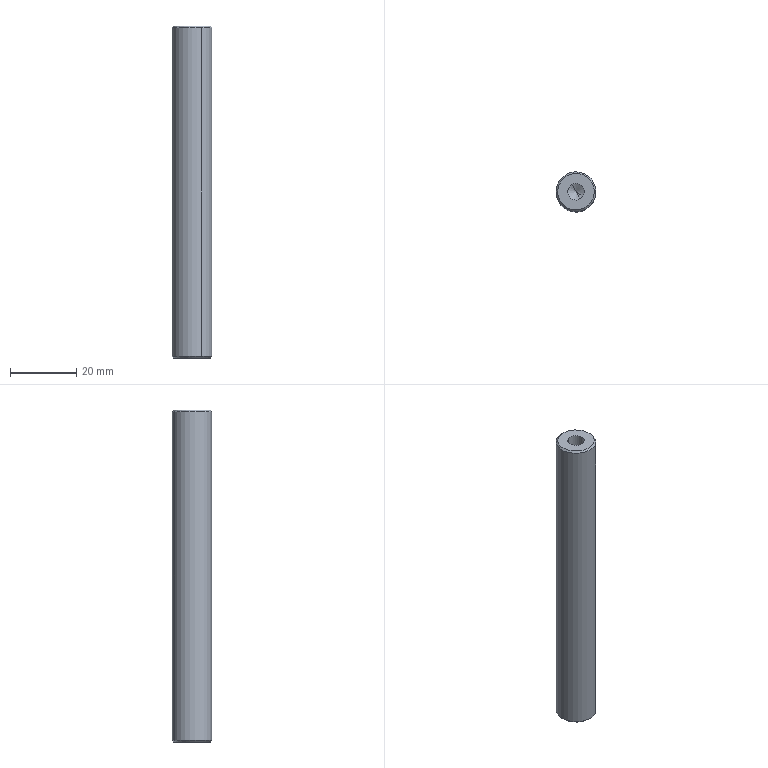Component | SolidWorks | A-C14LocatingMechanismGuidePost-1 | 1 solid | 12 faces | box 12 x 12 x 100 mm | volume 10996 mm3 | cone 6 | cylinder 4 | plane 2 | commonest cylinder face diameters 5 x2 12 x2
build123d program:
from build123d import *

# Parameters (mm, degrees)
SKETCH1_R             = 6
EXTRUDE1_DEPTH        = 100
CHAMFER1_SIZE         = 0.5
M6_TAPPED_HOLE1_D     = 5
M6_TAPPED_HOLE1_DEPTH = 15
M6_TAPPED_HOLE1_TIP   = 1.502


with BuildPart() as part:
    # Sketch1 → Extrude1 (new body)
    with BuildSketch(Plane.XY):
        Circle(SKETCH1_R)
    extrude(amount=EXTRUDE1_DEPTH)

    # Chamfer1
    chamfer1_edges = [part.edges().sort_by_distance(p)[0] for p in [
        (-6, 0, 0),
        (-6, 0, 100),
    ]]
    chamfer(chamfer1_edges, length=CHAMFER1_SIZE)

    # M6 Tapped Hole1
    with Locations(Plane(origin=(0, 0, 0), x_dir=(-1, 0, 0), z_dir=(0, 0, -1))):
        with Locations((0, 0)):
            Hole(M6_TAPPED_HOLE1_D / 2, depth=M6_TAPPED_HOLE1_DEPTH)
            with Locations((0, 0, -(M6_TAPPED_HOLE1_DEPTH + M6_TAPPED_HOLE1_TIP / 2))):  # 118° drill point
                Cone(0, M6_TAPPED_HOLE1_D / 2, M6_TAPPED_HOLE1_TIP, mode=Mode.SUBTRACT)


solid = part.part

# Placed as in the assembly
solid = solid.moved(Location((-53.181, -42.432, 18), (180, 0, 0)))
STEP:
#1=COLOUR_RGB('',0.7922,0.8196,0.9333);
#2=FILL_AREA_STYLE_COLOUR('',#1);
#3=FILL_AREA_STYLE('',(#2));
#4=SURFACE_STYLE_FILL_AREA(#3);
#5=SURFACE_SIDE_STYLE('',(#4));
#6=SURFACE_STYLE_USAGE(.BOTH.,#5);
#7=PRESENTATION_STYLE_ASSIGNMENT((#6));
#8=CARTESIAN_POINT('',(-2.142,-1.585,0.1181));
#9=VERTEX_POINT('',#8);
#10=CARTESIAN_POINT('',(-2.046,-1.757,0.1181));
#11=VERTEX_POINT('',#10);
#12=CARTESIAN_POINT('',(-2.094,-1.671,0.1181));
#13=DIRECTION('',(-0.,0.,1.));
#14=DIRECTION('',(0.4859,-0.874,0.));
#15=AXIS2_PLACEMENT_3D('',#12,#13,#14);
#16=CIRCLE('',#15,0.09843);
#17=EDGE_CURVE('',#9,#11,#16,.T.);
#18=ORIENTED_EDGE('',*,*,#17,.F.);
#19=CARTESIAN_POINT('',(-2.142,-1.585,0.7087));
#20=VERTEX_POINT('',#19);
#21=CARTESIAN_POINT('',(-2.142,-1.585,0.7087));
#22=DIRECTION('',(-0.,0.,1.));
#23=VECTOR('',#22,39.37);
#24=LINE('',#21,#23);
#25=EDGE_CURVE('',#9,#20,#24,.T.);
#26=ORIENTED_EDGE('',*,*,#25,.T.);
#27=CARTESIAN_POINT('',(-2.046,-1.757,0.7087));
#28=VERTEX_POINT('',#27);
#29=CARTESIAN_POINT('',(-2.094,-1.671,0.7087));
#30=DIRECTION('',(-0.,0.,1.));
#31=DIRECTION('',(0.4859,-0.874,0.));
#32=AXIS2_PLACEMENT_3D('',#29,#30,#31);
#33=CIRCLE('',#32,0.09843);
#34=EDGE_CURVE('',#20,#28,#33,.T.);
#35=ORIENTED_EDGE('',*,*,#34,.T.);
#36=CARTESIAN_POINT('',(-2.046,-1.757,0.7087));
#37=DIRECTION('',(-0.,0.,1.));
#38=VECTOR('',#37,39.37);
#39=LINE('',#36,#38);
#40=EDGE_CURVE('',#11,#28,#39,.T.);
#41=ORIENTED_EDGE('',*,*,#40,.F.);
#42=EDGE_LOOP('',(#18,#26,#35,#41));
#43=FACE_OUTER_BOUND('',#42,.T.);
#44=CARTESIAN_POINT('',(-2.094,-1.671,0.7087));
#45=DIRECTION('',(-0.,0.,1.));
#46=DIRECTION('',(0.4859,-0.874,0.));
#47=AXIS2_PLACEMENT_3D('',#44,#45,#46);
#48=CYLINDRICAL_SURFACE('',#47,0.09843);
#49=ADVANCED_FACE('',(#43),#48,.F.);
#50=CARTESIAN_POINT('',(-2.094,-1.671,0.05897));
#51=VERTEX_POINT('',#50);
#52=CARTESIAN_POINT('',(-2.046,-1.757,0.1181));
#53=DIRECTION('',(0.4165,-0.7492,0.515));
#54=VECTOR('',#53,39.37);
#55=LINE('',#52,#54);
#56=EDGE_CURVE('',#51,#11,#55,.T.);
#57=ORIENTED_EDGE('',*,*,#56,.F.);
#58=CARTESIAN_POINT('',(-2.142,-1.585,0.1181));
#59=DIRECTION('',(-0.4165,0.7492,0.515));
#60=VECTOR('',#59,39.37);
#61=LINE('',#58,#60);
#62=EDGE_CURVE('',#51,#9,#61,.T.);
#63=ORIENTED_EDGE('',*,*,#62,.T.);
#64=ORIENTED_EDGE('',*,*,#17,.T.);
#65=EDGE_LOOP('',(#57,#63,#64));
#66=FACE_OUTER_BOUND('',#65,.T.);
#67=CARTESIAN_POINT('',(-2.094,-1.671,0.1181));
#68=DIRECTION('',(-0.,0.,1.));
#69=DIRECTION('',(0.4859,-0.874,0.));
#70=AXIS2_PLACEMENT_3D('',#67,#68,#69);
#71=CONICAL_SURFACE('',#70,0.09843,1.03);
#72=ADVANCED_FACE('',(#66),#71,.F.);
#73=CARTESIAN_POINT('',(-2.199,-1.481,-3.228));
#74=VERTEX_POINT('',#73);
#75=CARTESIAN_POINT('',(-1.989,-1.86,-3.228));
#76=VERTEX_POINT('',#75);
#77=CARTESIAN_POINT('',(-2.094,-1.671,-3.228));
#78=DIRECTION('',(0.,-0.,-1.));
#79=DIRECTION('',(-0.4859,0.874,0.));
#80=AXIS2_PLACEMENT_3D('',#77,#78,#79);
#81=CIRCLE('',#80,0.2165);
#82=EDGE_CURVE('',#74,#76,#81,.T.);
#83=ORIENTED_EDGE('',*,*,#82,.F.);
#84=CARTESIAN_POINT('',(-2.208,-1.464,-3.209));
#85=VERTEX_POINT('',#84);
#86=CARTESIAN_POINT('',(-2.199,-1.481,-3.228));
#87=DIRECTION('',(-0.3436,0.618,0.7071));
#88=VECTOR('',#87,39.37);
#89=LINE('',#86,#88);
#90=EDGE_CURVE('',#74,#85,#89,.T.);
#91=ORIENTED_EDGE('',*,*,#90,.T.);
#92=CARTESIAN_POINT('',(-1.979,-1.877,-3.209));
#93=VERTEX_POINT('',#92);
#94=CARTESIAN_POINT('',(-2.094,-1.671,-3.209));
#95=DIRECTION('',(-0.,0.,1.));
#96=DIRECTION('',(-0.4859,0.874,0.));
#97=AXIS2_PLACEMENT_3D('',#94,#95,#96);
#98=CIRCLE('',#97,0.2362);
#99=EDGE_CURVE('',#93,#85,#98,.T.);
#100=ORIENTED_EDGE('',*,*,#99,.F.);
#101=CARTESIAN_POINT('',(-1.989,-1.86,-3.228));
#102=DIRECTION('',(0.3436,-0.618,0.7071));
#103=VECTOR('',#102,39.37);
#104=LINE('',#101,#103);
#105=EDGE_CURVE('',#76,#93,#104,.T.);
#106=ORIENTED_EDGE('',*,*,#105,.F.);
#107=EDGE_LOOP('',(#83,#91,#100,#106));
#108=FACE_OUTER_BOUND('',#107,.T.);
#109=CARTESIAN_POINT('',(-2.094,-1.671,-3.228));
#110=DIRECTION('',(-0.,0.,1.));
#111=DIRECTION('',(0.4859,-0.874,0.));
#112=AXIS2_PLACEMENT_3D('',#109,#110,#111);
#113=CONICAL_SURFACE('',#112,0.2165,0.7854);
#114=ADVANCED_FACE('',(#108),#113,.T.);
#115=CARTESIAN_POINT('',(-1.989,-1.86,0.7087));
#116=VERTEX_POINT('',#115);
#117=CARTESIAN_POINT('',(-2.199,-1.481,0.7087));
#118=VERTEX_POINT('',#117);
#119=CARTESIAN_POINT('',(-2.094,-1.671,0.7087));
#120=DIRECTION('',(-0.,0.,1.));
#121=DIRECTION('',(-0.4859,0.874,0.));
#122=AXIS2_PLACEMENT_3D('',#119,#120,#121);
#123=CIRCLE('',#122,0.2165);
#124=EDGE_CURVE('',#116,#118,#123,.T.);
#125=ORIENTED_EDGE('',*,*,#124,.F.);
#126=CARTESIAN_POINT('',(-1.979,-1.877,0.689));
#127=VERTEX_POINT('',#126);
#128=CARTESIAN_POINT('',(-1.979,-1.877,0.689));
#129=DIRECTION('',(0.3436,-0.618,-0.7071));
#130=VECTOR('',#129,39.37);
#131=LINE('',#128,#130);
#132=EDGE_CURVE('',#116,#127,#131,.T.);
#133=ORIENTED_EDGE('',*,*,#132,.T.);
#134=CARTESIAN_POINT('',(-2.208,-1.464,0.689));
#135=VERTEX_POINT('',#134);
#136=CARTESIAN_POINT('',(-2.094,-1.671,0.689));
#137=DIRECTION('',(0.,-0.,-1.));
#138=DIRECTION('',(-0.4859,0.874,0.));
#139=AXIS2_PLACEMENT_3D('',#136,#137,#138);
#140=CIRCLE('',#139,0.2362);
#141=EDGE_CURVE('',#135,#127,#140,.T.);
#142=ORIENTED_EDGE('',*,*,#141,.F.);
#143=CARTESIAN_POINT('',(-2.208,-1.464,0.689));
#144=DIRECTION('',(-0.3436,0.618,-0.7071));
#145=VECTOR('',#144,39.37);
#146=LINE('',#143,#145);
#147=EDGE_CURVE('',#118,#135,#146,.T.);
#148=ORIENTED_EDGE('',*,*,#147,.F.);
#149=EDGE_LOOP('',(#125,#133,#142,#148));
#150=FACE_OUTER_BOUND('',#149,.T.);
#151=CARTESIAN_POINT('',(-2.094,-1.671,0.689));
#152=DIRECTION('',(0.,-0.,-1.));
#153=DIRECTION('',(-0.4859,0.874,0.));
#154=AXIS2_PLACEMENT_3D('',#151,#152,#153);
#155=CONICAL_SURFACE('',#154,0.2362,0.7854);
#156=ADVANCED_FACE('',(#150),#155,.T.);
#157=ORIENTED_EDGE('',*,*,#99,.T.);
#158=CARTESIAN_POINT('',(-2.208,-1.464,-3.228));
#159=DIRECTION('',(-0.,0.,1.));
#160=VECTOR('',#159,39.37);
#161=LINE('',#158,#160);
#162=EDGE_CURVE('',#85,#135,#161,.T.);
#163=ORIENTED_EDGE('',*,*,#162,.T.);
#164=ORIENTED_EDGE('',*,*,#141,.T.);
#165=CARTESIAN_POINT('',(-1.979,-1.877,-3.228));
#166=DIRECTION('',(-0.,0.,1.));
#167=VECTOR('',#166,39.37);
#168=LINE('',#165,#167);
#169=EDGE_CURVE('',#93,#127,#168,.T.);
#170=ORIENTED_EDGE('',*,*,#169,.F.);
#171=EDGE_LOOP('',(#157,#163,#164,#170));
#172=FACE_OUTER_BOUND('',#171,.T.);
#173=CARTESIAN_POINT('',(-2.094,-1.671,-3.228));
#174=DIRECTION('',(-0.,0.,1.));
#175=DIRECTION('',(0.4859,-0.874,0.));
#176=AXIS2_PLACEMENT_3D('',#173,#174,#175);
#177=CYLINDRICAL_SURFACE('',#176,0.2362);
#178=ADVANCED_FACE('',(#172),#177,.T.);
#179=ORIENTED_EDGE('',*,*,#162,.F.);
#180=CARTESIAN_POINT('',(-2.094,-1.671,-3.209));
#181=DIRECTION('',(-0.,0.,1.));
#182=DIRECTION('',(-0.4859,0.874,0.));
#183=AXIS2_PLACEMENT_3D('',#180,#181,#182);
#184=CIRCLE('',#183,0.2362);
#185=EDGE_CURVE('',#85,#93,#184,.T.);
#186=ORIENTED_EDGE('',*,*,#185,.T.);
#187=ORIENTED_EDGE('',*,*,#169,.T.);
#188=CARTESIAN_POINT('',(-2.094,-1.671,0.689));
#189=DIRECTION('',(0.,-0.,-1.));
#190=DIRECTION('',(-0.4859,0.874,0.));
#191=AXIS2_PLACEMENT_3D('',#188,#189,#190);
#192=CIRCLE('',#191,0.2362);
#193=EDGE_CURVE('',#127,#135,#192,.T.);
#194=ORIENTED_EDGE('',*,*,#193,.T.);
#195=EDGE_LOOP('',(#179,#186,#187,#194));
#196=FACE_OUTER_BOUND('',#195,.T.);
#197=CARTESIAN_POINT('',(-2.094,-1.671,-3.228));
#198=DIRECTION('',(-0.,0.,1.));
#199=DIRECTION('',(0.4859,-0.874,0.));
#200=AXIS2_PLACEMENT_3D('',#197,#198,#199);
#201=CYLINDRICAL_SURFACE('',#200,0.2362);
#202=ADVANCED_FACE('',(#196),#201,.T.);
#203=CARTESIAN_POINT('',(-2.094,-1.671,-3.228));
#204=DIRECTION('',(0.,-0.,-1.));
#205=DIRECTION('',(-0.4859,0.874,0.));
#206=AXIS2_PLACEMENT_3D('',#203,#204,#205);
#207=CIRCLE('',#206,0.2165);
#208=EDGE_CURVE('',#76,#74,#207,.T.);
#209=ORIENTED_EDGE('',*,*,#208,.T.);
#210=ORIENTED_EDGE('',*,*,#82,.T.);
#211=EDGE_LOOP('',(#209,#210));
#212=FACE_OUTER_BOUND('',#211,.T.);
#213=CARTESIAN_POINT('',(-2.094,-1.671,-3.228));
#214=DIRECTION('',(0.,-0.,-1.));
#215=DIRECTION('',(-0.4859,0.874,-0.));
#216=AXIS2_PLACEMENT_3D('',#213,#214,#215);
#217=PLANE('',#216);
#218=ADVANCED_FACE('',(#212),#217,.T.);
#219=CARTESIAN_POINT('',(-2.094,-1.671,0.7087));
#220=DIRECTION('',(-0.,0.,1.));
#221=DIRECTION('',(0.4859,-0.874,0.));
#222=AXIS2_PLACEMENT_3D('',#219,#220,#221);
#223=CIRCLE('',#222,0.09843);
#224=EDGE_CURVE('',#28,#20,#223,.T.);
#225=ORIENTED_EDGE('',*,*,#224,.F.);
#226=ORIENTED_EDGE('',*,*,#34,.F.);
#227=EDGE_LOOP('',(#225,#226));
#228=FACE_BOUND('',#227,.T.);
#229=CARTESIAN_POINT('',(-2.094,-1.671,0.7087));
#230=DIRECTION('',(-0.,0.,1.));
#231=DIRECTION('',(-0.4859,0.874,0.));
#232=AXIS2_PLACEMENT_3D('',#229,#230,#231);
#233=CIRCLE('',#232,0.2165);
#234=EDGE_CURVE('',#118,#116,#233,.T.);
#235=ORIENTED_EDGE('',*,*,#234,.T.);
#236=ORIENTED_EDGE('',*,*,#124,.T.);
#237=EDGE_LOOP('',(#235,#236));
#238=FACE_OUTER_BOUND('',#237,.T.);
#239=CARTESIAN_POINT('',(-2.094,-1.671,0.7087));
#240=DIRECTION('',(0.,-0.,-1.));
#241=DIRECTION('',(-0.4859,0.874,-0.));
#242=AXIS2_PLACEMENT_3D('',#239,#240,#241);
#243=PLANE('',#242);
#244=ADVANCED_FACE('',(#228,#238),#243,.F.);
#245=ORIENTED_EDGE('',*,*,#132,.F.);
#246=ORIENTED_EDGE('',*,*,#234,.F.);
#247=ORIENTED_EDGE('',*,*,#147,.T.);
#248=ORIENTED_EDGE('',*,*,#193,.F.);
#249=EDGE_LOOP('',(#245,#246,#247,#248));
#250=FACE_OUTER_BOUND('',#249,.T.);
#251=CARTESIAN_POINT('',(-2.094,-1.671,0.689));
#252=DIRECTION('',(0.,-0.,-1.));
#253=DIRECTION('',(-0.4859,0.874,0.));
#254=AXIS2_PLACEMENT_3D('',#251,#252,#253);
#255=CONICAL_SURFACE('',#254,0.2362,0.7854);
#256=ADVANCED_FACE('',(#250),#255,.T.);
#257=ORIENTED_EDGE('',*,*,#90,.F.);
#258=ORIENTED_EDGE('',*,*,#208,.F.);
#259=ORIENTED_EDGE('',*,*,#105,.T.);
#260=ORIENTED_EDGE('',*,*,#185,.F.);
#261=EDGE_LOOP('',(#257,#258,#259,#260));
#262=FACE_OUTER_BOUND('',#261,.T.);
#263=CARTESIAN_POINT('',(-2.094,-1.671,-3.228));
#264=DIRECTION('',(-0.,0.,1.));
#265=DIRECTION('',(0.4859,-0.874,0.));
#266=AXIS2_PLACEMENT_3D('',#263,#264,#265);
#267=CONICAL_SURFACE('',#266,0.2165,0.7854);
#268=ADVANCED_FACE('',(#262),#267,.T.);
#269=ORIENTED_EDGE('',*,*,#62,.F.);
#270=ORIENTED_EDGE('',*,*,#56,.T.);
#271=CARTESIAN_POINT('',(-2.094,-1.671,0.1181));
#272=DIRECTION('',(-0.,0.,1.));
#273=DIRECTION('',(0.4859,-0.874,0.));
#274=AXIS2_PLACEMENT_3D('',#271,#272,#273);
#275=CIRCLE('',#274,0.09843);
#276=EDGE_CURVE('',#11,#9,#275,.T.);
#277=ORIENTED_EDGE('',*,*,#276,.T.);
#278=EDGE_LOOP('',(#269,#270,#277));
#279=FACE_OUTER_BOUND('',#278,.T.);
#280=CARTESIAN_POINT('',(-2.094,-1.671,0.1181));
#281=DIRECTION('',(-0.,0.,1.));
#282=DIRECTION('',(0.4859,-0.874,0.));
#283=AXIS2_PLACEMENT_3D('',#280,#281,#282);
#284=CONICAL_SURFACE('',#283,0.09843,1.03);
#285=ADVANCED_FACE('',(#279),#284,.F.);
#286=ORIENTED_EDGE('',*,*,#25,.F.);
#287=ORIENTED_EDGE('',*,*,#276,.F.);
#288=ORIENTED_EDGE('',*,*,#40,.T.);
#289=ORIENTED_EDGE('',*,*,#224,.T.);
#290=EDGE_LOOP('',(#286,#287,#288,#289));
#291=FACE_OUTER_BOUND('',#290,.T.);
#292=CARTESIAN_POINT('',(-2.094,-1.671,0.7087));
#293=DIRECTION('',(-0.,0.,1.));
#294=DIRECTION('',(0.4859,-0.874,0.));
#295=AXIS2_PLACEMENT_3D('',#292,#293,#294);
#296=CYLINDRICAL_SURFACE('',#295,0.09843);
#297=ADVANCED_FACE('',(#291),#296,.F.);
#298=CLOSED_SHELL('',(#49,#72,#114,#156,#178,#202,#218,#244,#256,#268,#285,#297));
#299=MANIFOLD_SOLID_BREP('',#298);
#300=STYLED_ITEM('',(#7),#299);
#301=PRESENTATION_LAYER_ASSIGNMENT('','',(#300));
#302=(LENGTH_UNIT()NAMED_UNIT(*)SI_UNIT($,.METRE.));
#303=LENGTH_MEASURE_WITH_UNIT(LENGTH_MEASURE(0.0254),#302);
#304=DIMENSIONAL_EXPONENTS(1.,0.,0.,0.,0.,0.,0.);
#305=(CONVERSION_BASED_UNIT('',#303)LENGTH_UNIT()NAMED_UNIT(#304));
#306=UNCERTAINTY_MEASURE_WITH_UNIT(LENGTH_MEASURE(0.00001),#305,'','');
#307=(NAMED_UNIT(*)PLANE_ANGLE_UNIT()SI_UNIT($,.RADIAN.));
#308=(NAMED_UNIT(*)SI_UNIT($,.STERADIAN.)SOLID_ANGLE_UNIT());
#309=(GEOMETRIC_REPRESENTATION_CONTEXT(3)GLOBAL_UNCERTAINTY_ASSIGNED_CONTEXT((#306))GLOBAL_UNIT_ASSIGNED_CONTEXT((#305,#307,#308))REPRESENTATION_CONTEXT('',''));
#310=MECHANICAL_DESIGN_GEOMETRIC_PRESENTATION_REPRESENTATION('',(#300),#309);
#311=CARTESIAN_POINT('',(0.,0.,0.));
#312=DIRECTION('',(0.,0.,1.));
#313=DIRECTION('',(1.,0.,0.));
#314=AXIS2_PLACEMENT_3D('',#311,#312,#313);
#315=(LENGTH_UNIT()NAMED_UNIT(*)SI_UNIT($,.METRE.));
#316=LENGTH_MEASURE_WITH_UNIT(LENGTH_MEASURE(0.0254),#315);
#317=DIMENSIONAL_EXPONENTS(1.,0.,0.,0.,0.,0.,0.);
#318=(CONVERSION_BASED_UNIT('',#316)LENGTH_UNIT()NAMED_UNIT(#317));
#319=UNCERTAINTY_MEASURE_WITH_UNIT(LENGTH_MEASURE(0.00001),#318,'','');
#320=(NAMED_UNIT(*)PLANE_ANGLE_UNIT()SI_UNIT($,.RADIAN.));
#321=(NAMED_UNIT(*)SI_UNIT($,.STERADIAN.)SOLID_ANGLE_UNIT());
#322=(GEOMETRIC_REPRESENTATION_CONTEXT(3)GLOBAL_UNCERTAINTY_ASSIGNED_CONTEXT((#319))GLOBAL_UNIT_ASSIGNED_CONTEXT((#318,#320,#321))REPRESENTATION_CONTEXT('',''));
#323=ADVANCED_BREP_SHAPE_REPRESENTATION('',(#299,#314),#322);